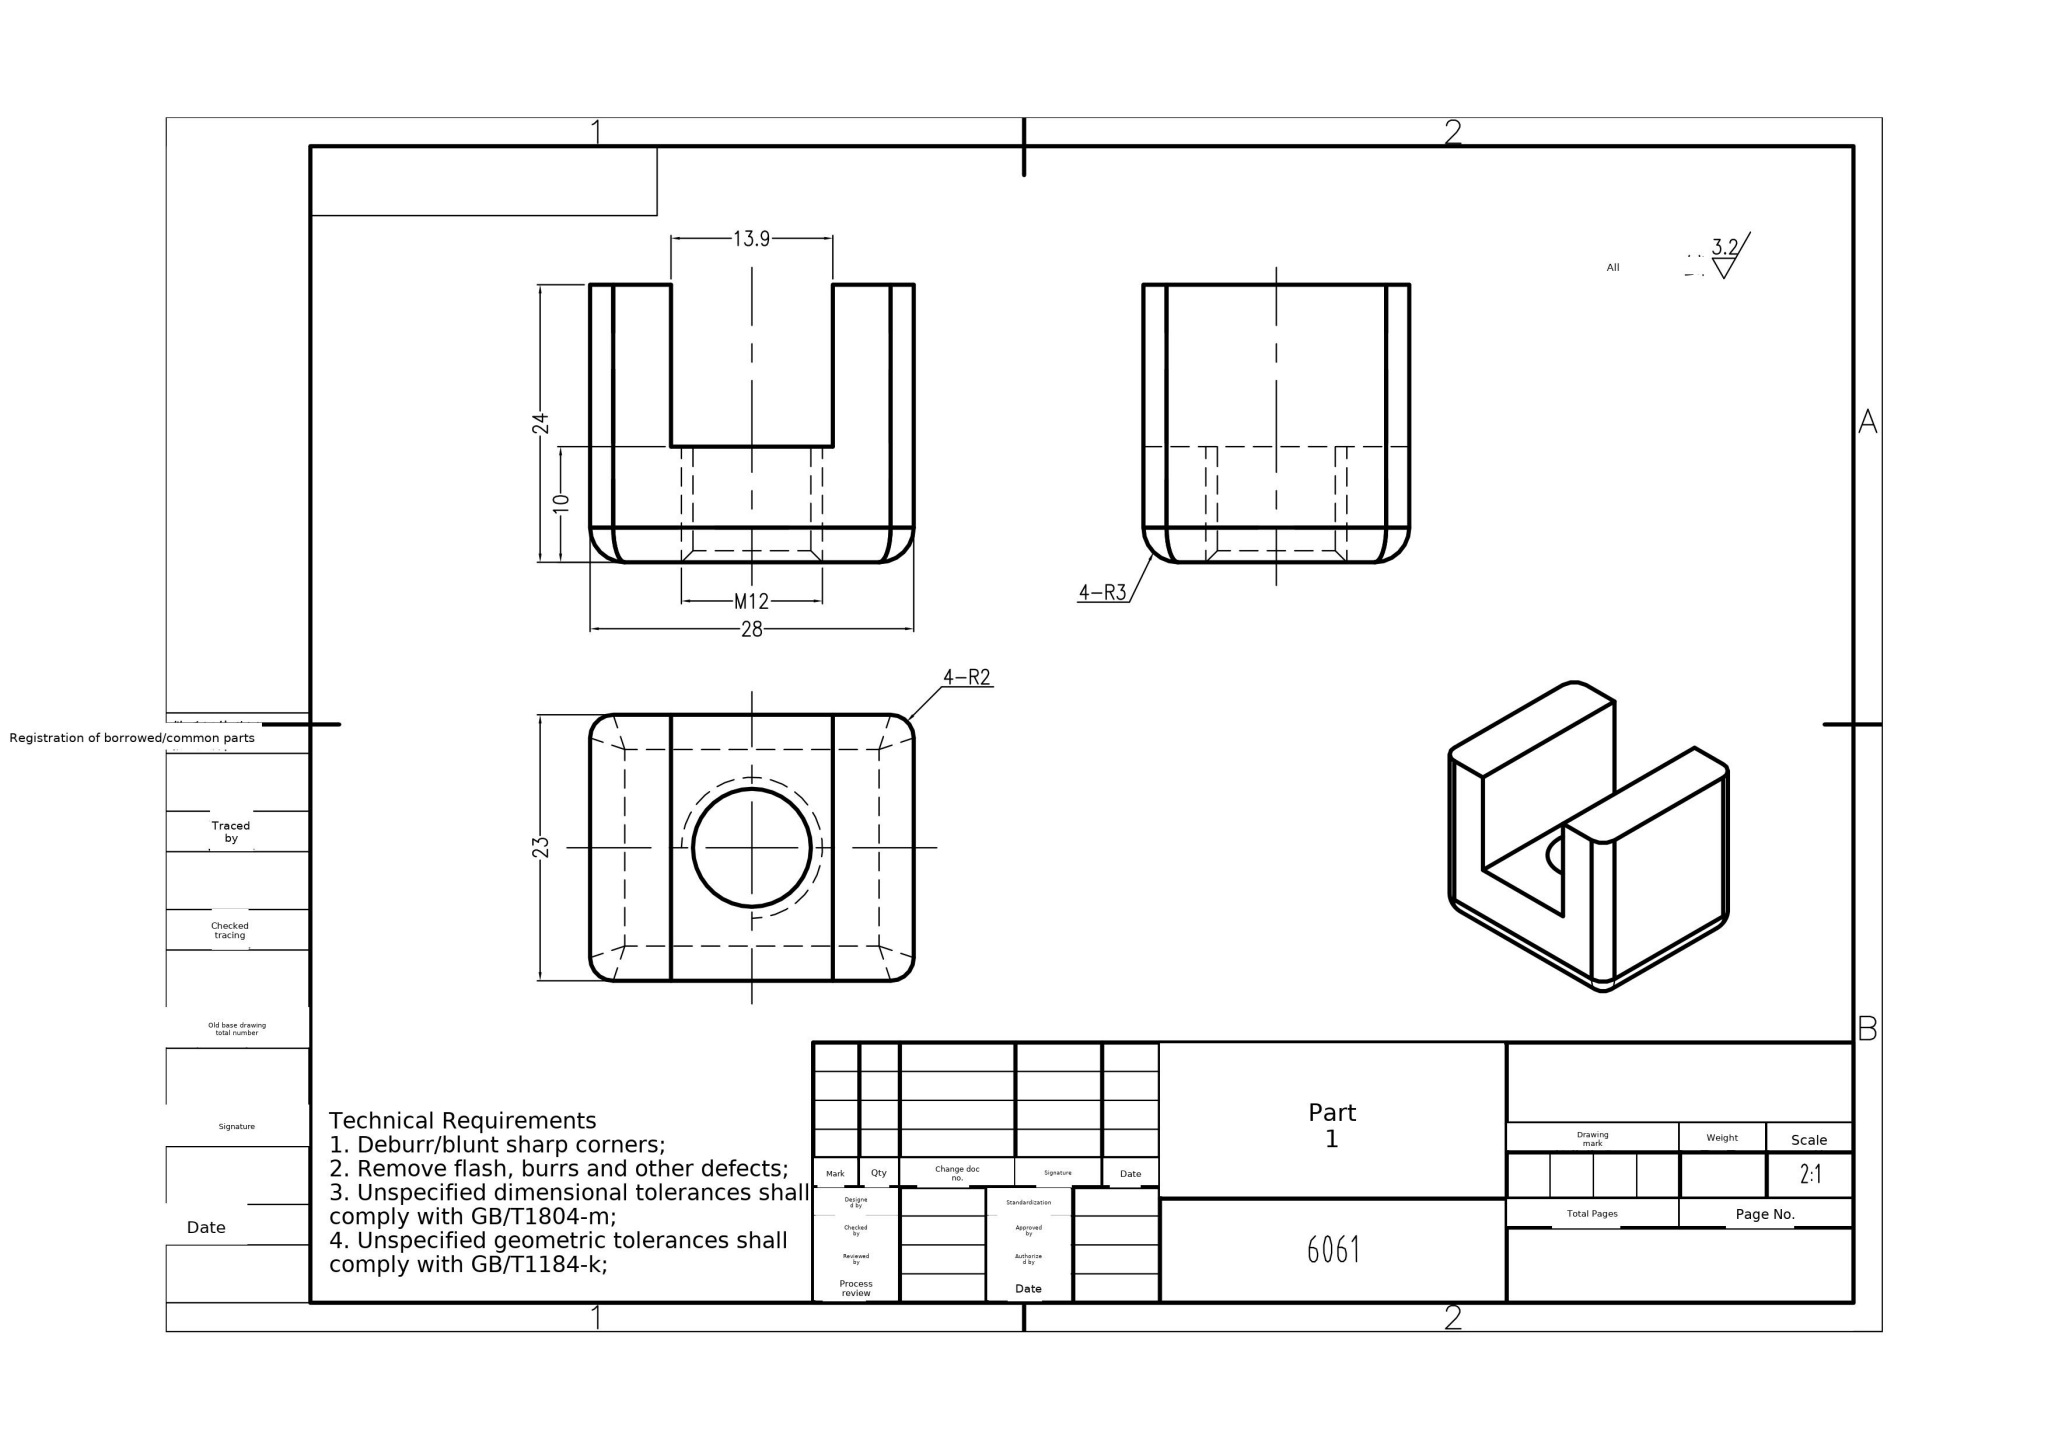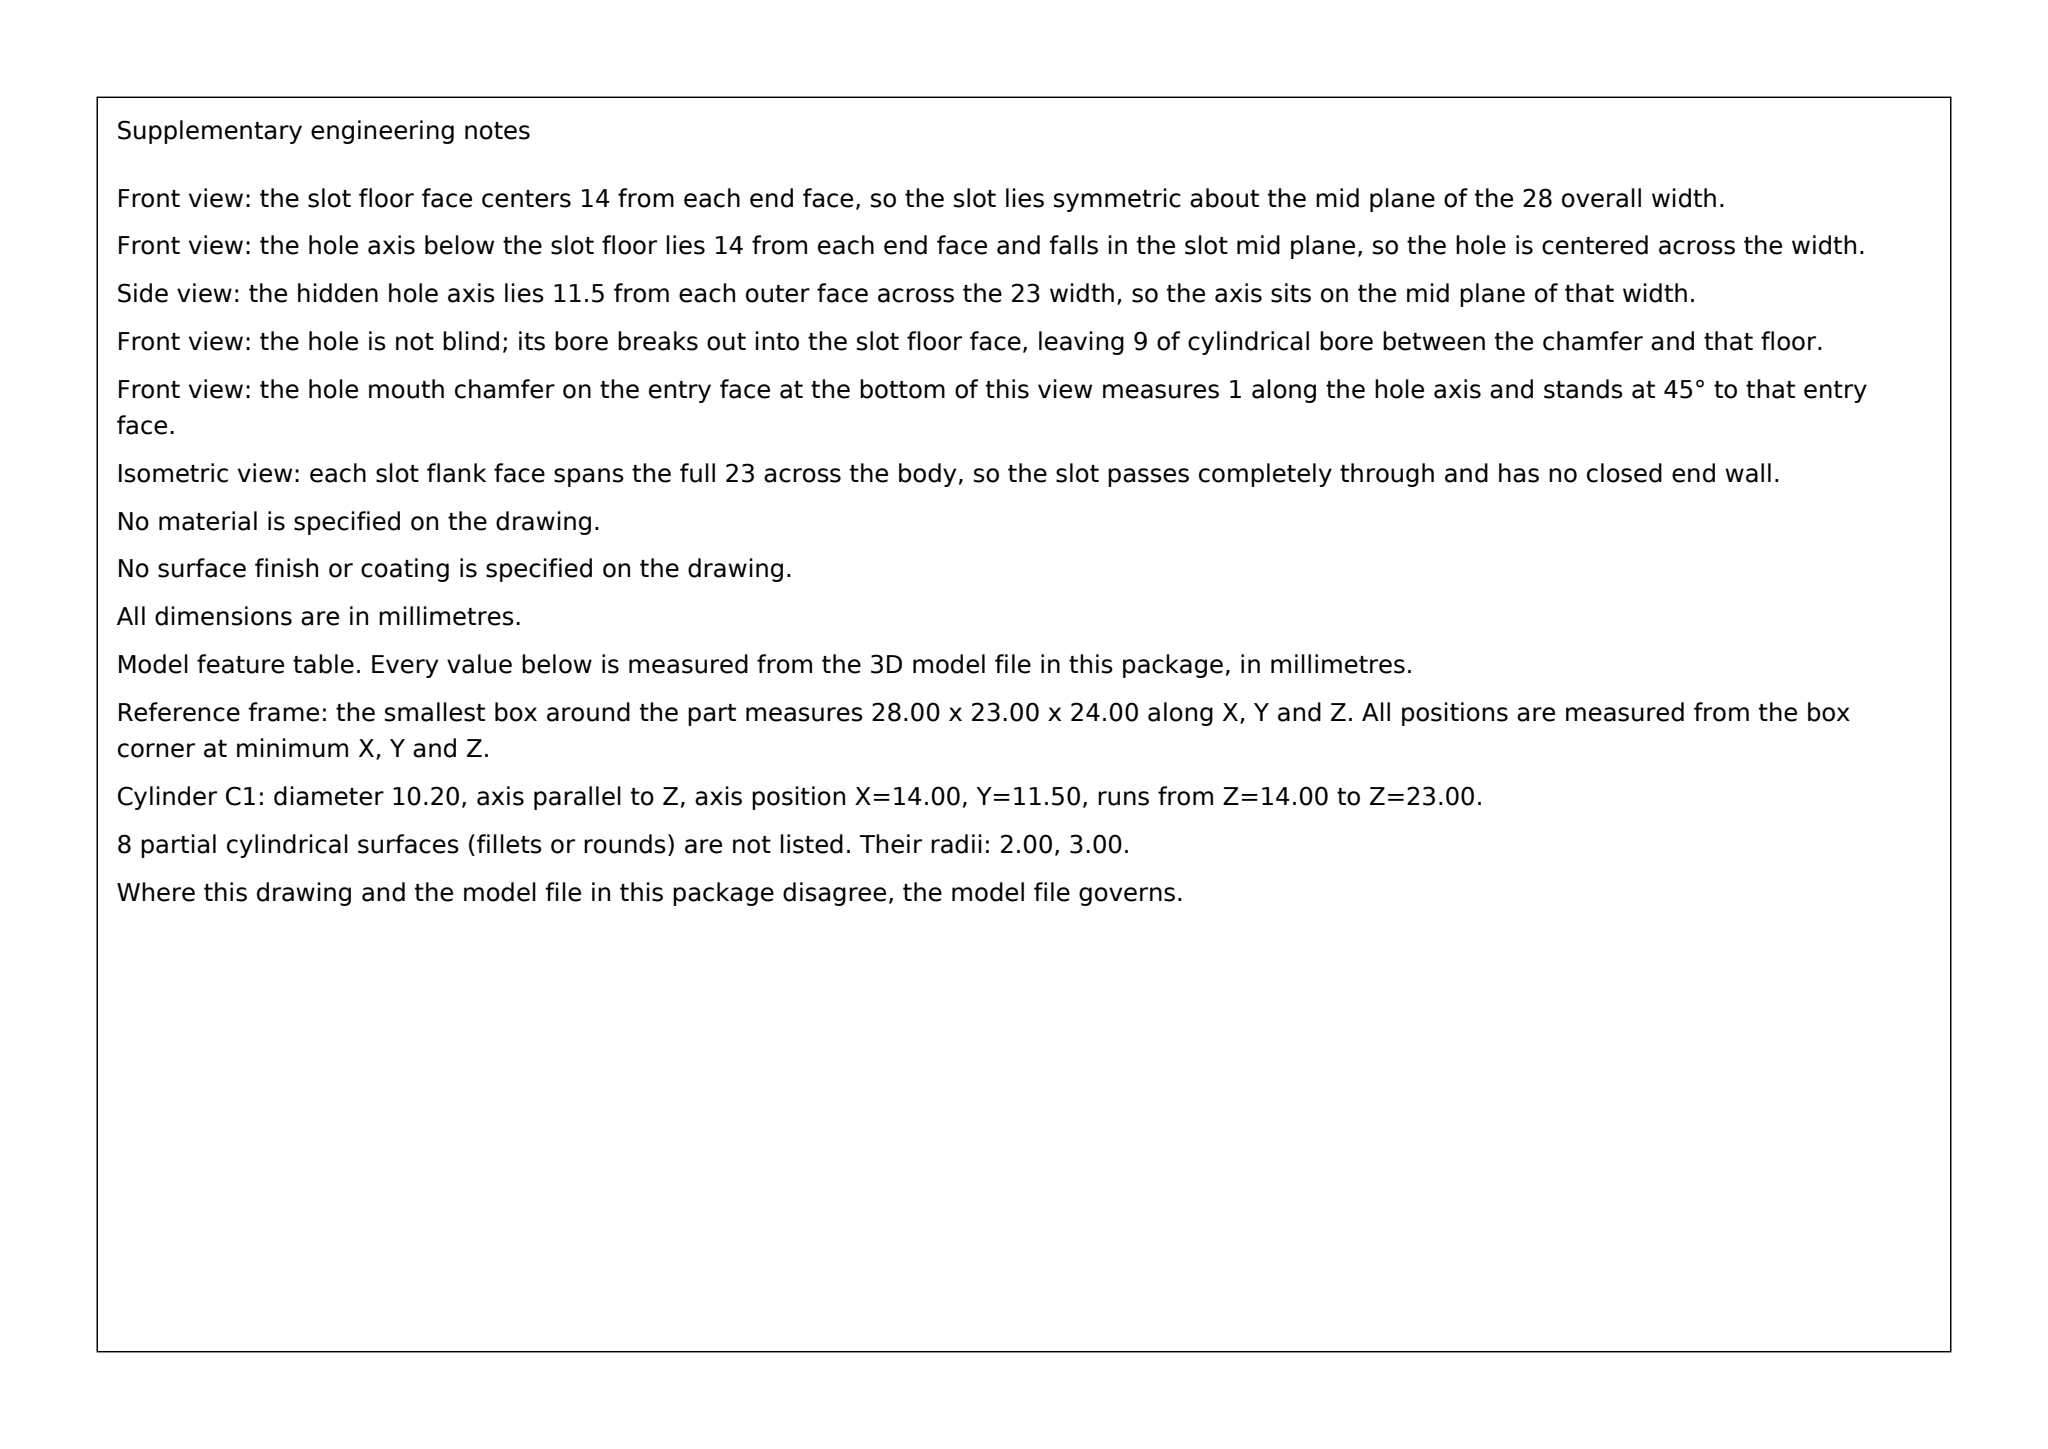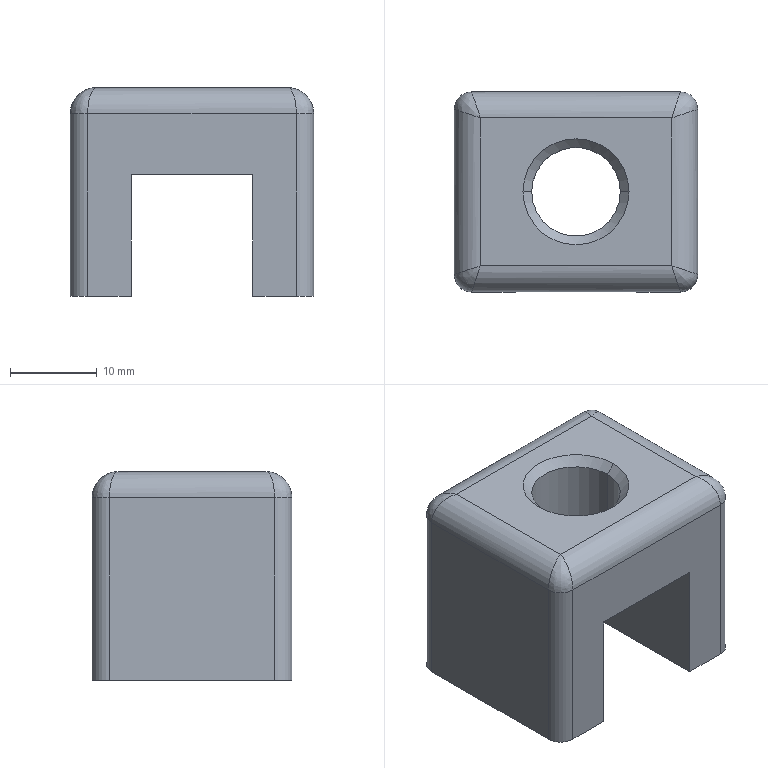Part | SolidWorks | mm | material 6061 | 1 solid | 26 faces | box 28 x 23 x 24 mm | volume 9848 mm3 | cylinder 10 | plane 10 | spline 4 | cone 2 | commonest cylinder face diameters 6 x4 4 x4 10.2 x2
Drawing notes:
M12 DP 9 FROM SLOT FLOOR; Ø10.2 DRILL DP 10 (BLIND) | from the solid: hole/bore Ø10.2 axis z at (14.0,11.5) from 14.0 to 23.0 = 9 deep from slot floor plane z=14; 90° cone drill point z=23-24 adds 1 -> drill 10
CHAMFER CALLOUT READS 1-C1 AT M12 HOLE MOUTH, 1 PLACE | from the solid: only one tapped feature in STEP (single Ø10.2 bore at x14, y11.5); no other chamfered edges (inclined_planes empty)